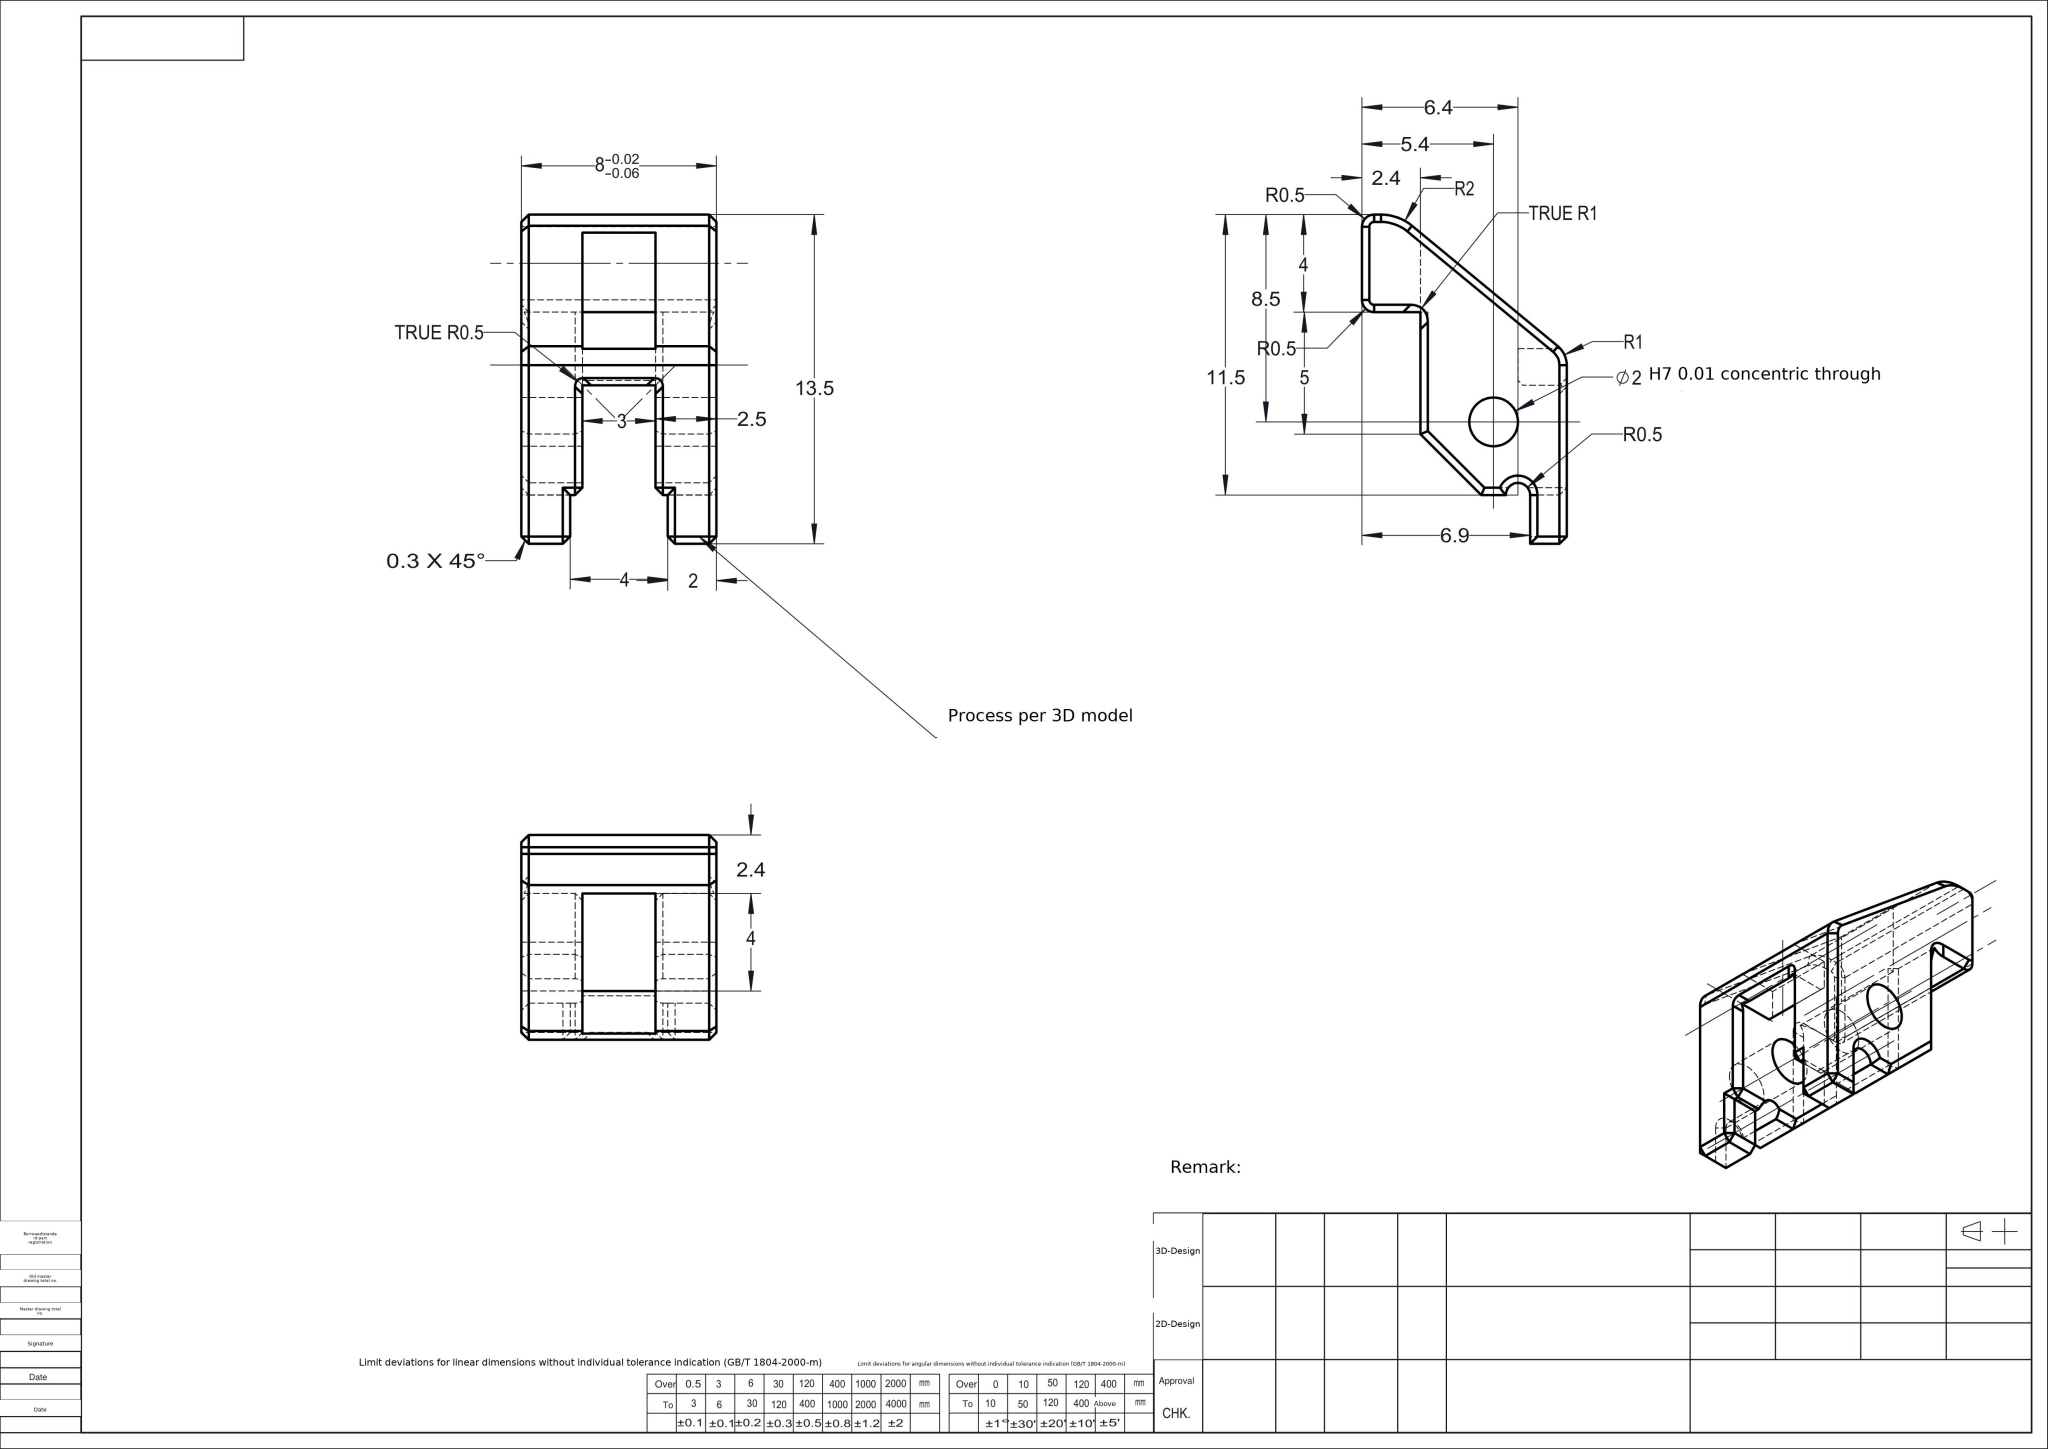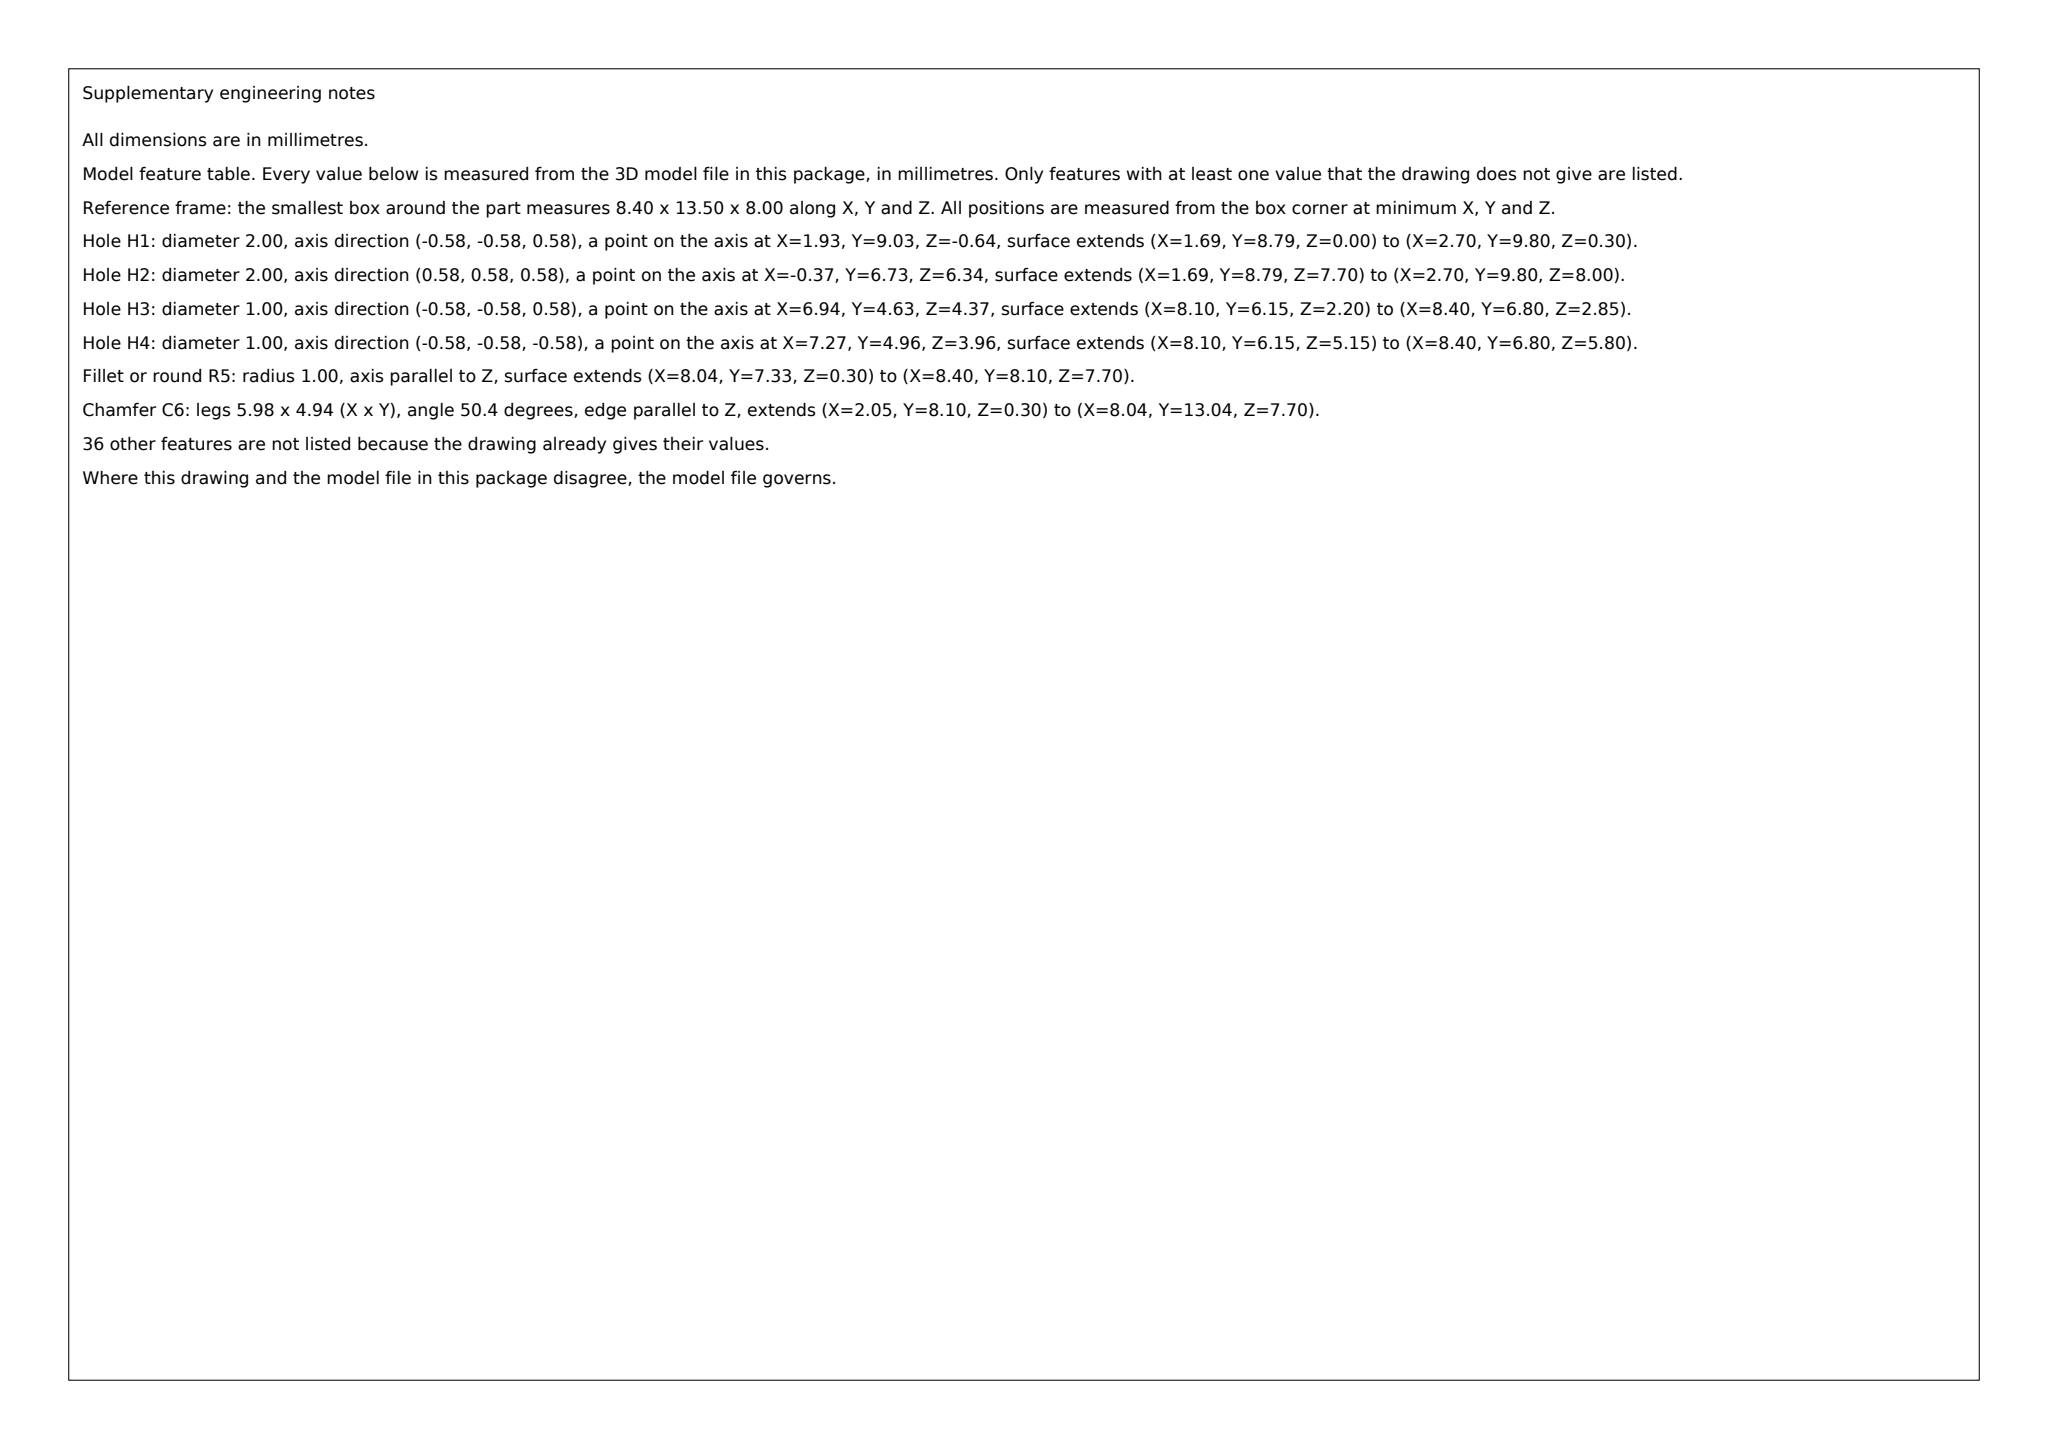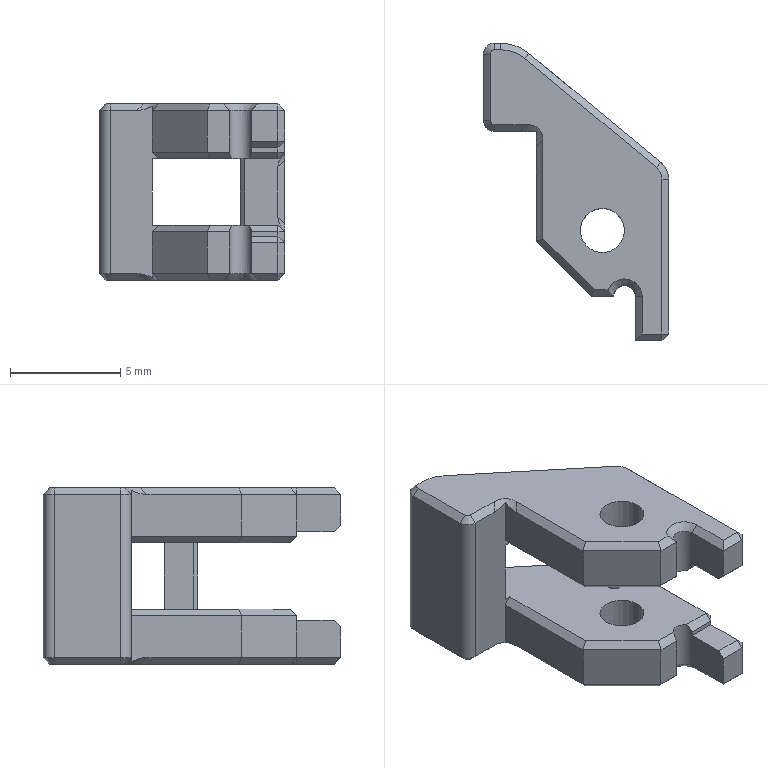Part | SolidWorks | mm | 1 solid | 97 faces | box 8.4 x 13.5 x 8 mm | volume 303 mm3 | plane 73 | cylinder 14 | cone 10 | commonest cylinder face diameters 2 x7 1 x6 4 x1